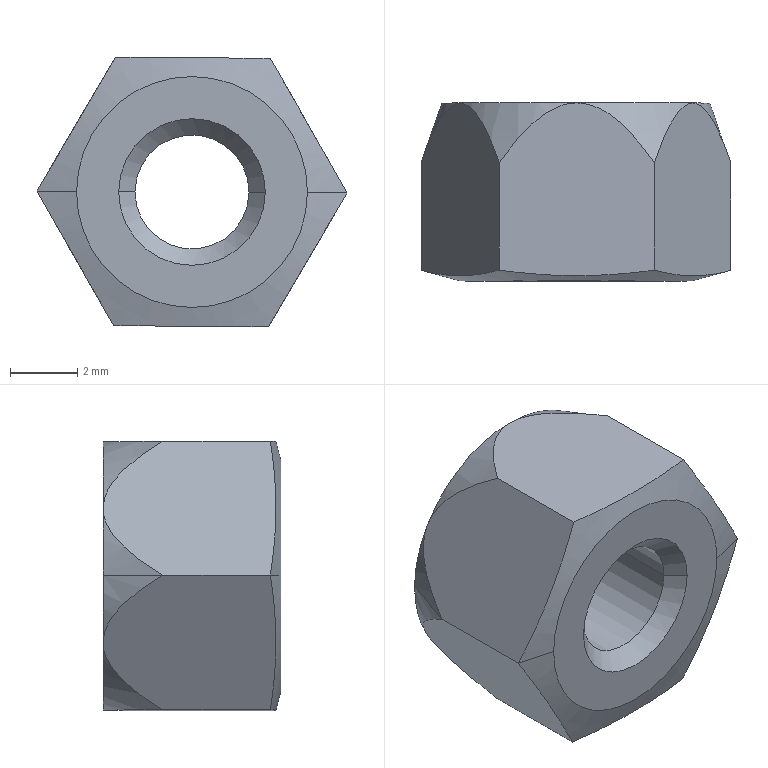Component | SolidWorks | prevailing torque all-metal 1 gb-4 | 1 solid | 21 faces | box 9.24 x 5.3 x 8.03 mm | volume 239 mm3 | cone 11 | plane 8 | cylinder 2 | commonest cylinder face diameters 3.4 x2
STEP:
#1=COLOUR_RGB('',0.7922,0.8196,0.9333);
#2=FILL_AREA_STYLE_COLOUR('',#1);
#3=FILL_AREA_STYLE('',(#2));
#4=SURFACE_STYLE_FILL_AREA(#3);
#5=SURFACE_SIDE_STYLE('',(#4));
#6=SURFACE_STYLE_USAGE(.BOTH.,#5);
#7=PRESENTATION_STYLE_ASSIGNMENT((#6));
#8=CARTESIAN_POINT('',(0.2638,-0.3076,1.348));
#9=VERTEX_POINT('',#8);
#10=CARTESIAN_POINT('',(0.1299,-0.3076,1.349));
#11=VERTEX_POINT('',#10);
#12=CARTESIAN_POINT('',(0.1969,-0.3076,1.348));
#13=DIRECTION('',(0.,-1.,0.));
#14=DIRECTION('',(-1.,0.,0.006451));
#15=AXIS2_PLACEMENT_3D('',#12,#13,#14);
#16=CIRCLE('',#15,0.06693);
#17=EDGE_CURVE('',#9,#11,#16,.T.);
#18=ORIENTED_EDGE('',*,*,#17,.F.);
#19=CARTESIAN_POINT('',(0.2829,-0.3268,1.348));
#20=VERTEX_POINT('',#19);
#21=CARTESIAN_POINT('',(0.2829,-0.3268,1.348));
#22=DIRECTION('',(0.7071,-0.7071,-0.004562));
#23=VECTOR('',#22,39.37);
#24=LINE('',#21,#23);
#25=EDGE_CURVE('',#9,#20,#24,.T.);
#26=ORIENTED_EDGE('',*,*,#25,.T.);
#27=CARTESIAN_POINT('',(0.1108,-0.3268,1.349));
#28=VERTEX_POINT('',#27);
#29=CARTESIAN_POINT('',(0.1969,-0.3268,1.348));
#30=DIRECTION('',(0.,1.,0.));
#31=DIRECTION('',(-1.,0.,0.006451));
#32=AXIS2_PLACEMENT_3D('',#29,#30,#31);
#33=CIRCLE('',#32,0.08605);
#34=EDGE_CURVE('',#28,#20,#33,.T.);
#35=ORIENTED_EDGE('',*,*,#34,.F.);
#36=CARTESIAN_POINT('',(0.1108,-0.3268,1.349));
#37=DIRECTION('',(-0.7071,-0.7071,0.004562));
#38=VECTOR('',#37,39.37);
#39=LINE('',#36,#38);
#40=EDGE_CURVE('',#11,#28,#39,.T.);
#41=ORIENTED_EDGE('',*,*,#40,.F.);
#42=EDGE_LOOP('',(#18,#26,#35,#41));
#43=FACE_OUTER_BOUND('',#42,.T.);
#44=CARTESIAN_POINT('',(0.1969,-0.3268,1.348));
#45=DIRECTION('',(0.,-1.,0.));
#46=DIRECTION('',(-1.,0.,0.006451));
#47=AXIS2_PLACEMENT_3D('',#44,#45,#46);
#48=CONICAL_SURFACE('',#47,0.08605,0.7854);
#49=ADVANCED_FACE('',(#43),#48,.F.);
#50=ORIENTED_EDGE('',*,*,#17,.T.);
#51=CARTESIAN_POINT('',(0.1299,-0.1181,1.349));
#52=VERTEX_POINT('',#51);
#53=CARTESIAN_POINT('',(0.1299,-0.3268,1.349));
#54=DIRECTION('',(0.,1.,0.));
#55=VECTOR('',#54,39.37);
#56=LINE('',#53,#55);
#57=EDGE_CURVE('',#11,#52,#56,.T.);
#58=ORIENTED_EDGE('',*,*,#57,.T.);
#59=CARTESIAN_POINT('',(0.2638,-0.1181,1.348));
#60=VERTEX_POINT('',#59);
#61=CARTESIAN_POINT('',(0.1969,-0.1181,1.348));
#62=DIRECTION('',(0.,1.,0.));
#63=DIRECTION('',(1.,0.,-0.006451));
#64=AXIS2_PLACEMENT_3D('',#61,#62,#63);
#65=CIRCLE('',#64,0.06693);
#66=EDGE_CURVE('',#52,#60,#65,.T.);
#67=ORIENTED_EDGE('',*,*,#66,.T.);
#68=CARTESIAN_POINT('',(0.2638,-0.3268,1.348));
#69=DIRECTION('',(0.,1.,0.));
#70=VECTOR('',#69,39.37);
#71=LINE('',#68,#70);
#72=EDGE_CURVE('',#9,#60,#71,.T.);
#73=ORIENTED_EDGE('',*,*,#72,.F.);
#74=EDGE_LOOP('',(#50,#58,#67,#73));
#75=FACE_OUTER_BOUND('',#74,.T.);
#76=CARTESIAN_POINT('',(0.1969,-0.3268,1.348));
#77=DIRECTION('',(0.,1.,0.));
#78=DIRECTION('',(1.,0.,-0.006451));
#79=AXIS2_PLACEMENT_3D('',#76,#77,#78);
#80=CYLINDRICAL_SURFACE('',#79,0.06693);
#81=ADVANCED_FACE('',(#75),#80,.F.);
#82=CARTESIAN_POINT('',(0.03937,-0.1181,1.349));
#83=VERTEX_POINT('',#82);
#84=CARTESIAN_POINT('',(0.06098,-0.1181,1.428));
#85=VERTEX_POINT('',#84);
#86=CARTESIAN_POINT('',(0.1969,-0.1181,1.348));
#87=DIRECTION('',(0.,1.,0.));
#88=DIRECTION('',(-1.,0.,0.006451));
#89=AXIS2_PLACEMENT_3D('',#86,#87,#88);
#90=CIRCLE('',#89,0.1575);
#91=EDGE_CURVE('',#83,#85,#90,.T.);
#92=ORIENTED_EDGE('',*,*,#91,.F.);
#93=CARTESIAN_POINT('',(0.01501,-0.1882,1.35));
#94=VERTEX_POINT('',#93);
#95=CARTESIAN_POINT('',(0.03937,-0.1181,1.349));
#96=DIRECTION('',(-0.3284,-0.9446,0.002118));
#97=VECTOR('',#96,39.37);
#98=LINE('',#95,#97);
#99=EDGE_CURVE('',#83,#94,#98,.T.);
#100=ORIENTED_EDGE('',*,*,#99,.T.);
#101=CARTESIAN_POINT('',(0.01501,-0.1882,1.35));
#102=CARTESIAN_POINT('',(0.01787,-0.18,1.354));
#103=CARTESIAN_POINT('',(0.02086,-0.1721,1.36));
#104=CARTESIAN_POINT('',(0.0272,-0.1569,1.37));
#105=CARTESIAN_POINT('',(0.03056,-0.1496,1.376));
#106=CARTESIAN_POINT('',(0.03795,-0.1363,1.389));
#107=CARTESIAN_POINT('',(0.042,-0.1301,1.396));
#108=CARTESIAN_POINT('',(0.05094,-0.121,1.411));
#109=CARTESIAN_POINT('',(0.05593,-0.1181,1.419));
#110=CARTESIAN_POINT('',(0.06098,-0.1181,1.428));
#111=B_SPLINE_CURVE_WITH_KNOTS('',3,(#101,#102,#103,#104,#105,#106,#107,#108,#109,#110),.UNSPECIFIED.,.F.,.F.,(4,2,2,2,4),(0.00000024,0.000751,0.001502,0.002252,0.003003),.UNSPECIFIED.);
#112=EDGE_CURVE('',#94,#85,#111,.T.);
#113=ORIENTED_EDGE('',*,*,#112,.T.);
#114=EDGE_LOOP('',(#92,#100,#113));
#115=FACE_OUTER_BOUND('',#114,.T.);
#116=CARTESIAN_POINT('',(0.1969,-0.1181,1.348));
#117=DIRECTION('',(0.,-1.,-0.));
#118=DIRECTION('',(-1.,-0.,0.006451));
#119=AXIS2_PLACEMENT_3D('',#116,#117,#118);
#120=CONICAL_SURFACE('',#119,0.1575,0.3346);
#121=ADVANCED_FACE('',(#115),#120,.T.);
#122=CARTESIAN_POINT('',(0.06142,-0.3268,1.349));
#123=VERTEX_POINT('',#122);
#124=CARTESIAN_POINT('',(0.3323,-0.3268,1.348));
#125=VERTEX_POINT('',#124);
#126=CARTESIAN_POINT('',(0.1969,-0.3268,1.348));
#127=DIRECTION('',(0.,-1.,-0.));
#128=DIRECTION('',(-1.,0.,0.006451));
#129=AXIS2_PLACEMENT_3D('',#126,#127,#128);
#130=CIRCLE('',#129,0.1354);
#131=EDGE_CURVE('',#123,#125,#130,.T.);
#132=ORIENTED_EDGE('',*,*,#131,.F.);
#133=CARTESIAN_POINT('',(0.01501,-0.3143,1.35));
#134=VERTEX_POINT('',#133);
#135=CARTESIAN_POINT('',(0.01501,-0.3143,1.35));
#136=DIRECTION('',(-0.9659,0.2588,0.006231));
#137=VECTOR('',#136,39.37);
#138=LINE('',#135,#137);
#139=EDGE_CURVE('',#123,#134,#138,.T.);
#140=ORIENTED_EDGE('',*,*,#139,.T.);
#141=CARTESIAN_POINT('',(0.1049,-0.3143,1.192));
#142=VERTEX_POINT('',#141);
#143=CARTESIAN_POINT('',(0.01501,-0.3143,1.35));
#144=CARTESIAN_POINT('',(0.03,-0.3184,1.323));
#145=CARTESIAN_POINT('',(0.05996,-0.3233,1.271));
#146=CARTESIAN_POINT('',(0.08993,-0.3184,1.218));
#147=CARTESIAN_POINT('',(0.1049,-0.3143,1.192));
#148=B_SPLINE_CURVE_WITH_KNOTS('',3,(#143,#144,#145,#146,#147),.UNSPECIFIED.,.F.,.F.,(4,1,4),(0.00000023,0.00231,0.004619),.UNSPECIFIED.);
#149=EDGE_CURVE('',#134,#142,#148,.T.);
#150=ORIENTED_EDGE('',*,*,#149,.T.);
#151=CARTESIAN_POINT('',(0.2868,-0.3143,1.19));
#152=VERTEX_POINT('',#151);
#153=CARTESIAN_POINT('',(0.1049,-0.3143,1.192));
#154=CARTESIAN_POINT('',(0.12,-0.3164,1.191));
#155=CARTESIAN_POINT('',(0.1353,-0.318,1.191));
#156=CARTESIAN_POINT('',(0.1657,-0.3203,1.191));
#157=CARTESIAN_POINT('',(0.1808,-0.3209,1.191));
#158=CARTESIAN_POINT('',(0.2263,-0.3209,1.191));
#159=CARTESIAN_POINT('',(0.2566,-0.3184,1.191));
#160=CARTESIAN_POINT('',(0.2868,-0.3143,1.19));
#161=B_SPLINE_CURVE_WITH_KNOTS('',3,(#153,#154,#155,#156,#157,#158,#159,#160),.UNSPECIFIED.,.F.,.F.,(4,2,2,4),(0.003852,0.005015,0.006177,0.008501),.UNSPECIFIED.);
#162=EDGE_CURVE('',#142,#152,#161,.T.);
#163=ORIENTED_EDGE('',*,*,#162,.T.);
#164=CARTESIAN_POINT('',(0.3787,-0.3143,1.347));
#165=VERTEX_POINT('',#164);
#166=CARTESIAN_POINT('',(0.2868,-0.3143,1.19));
#167=CARTESIAN_POINT('',(0.3021,-0.3184,1.217));
#168=CARTESIAN_POINT('',(0.3327,-0.3233,1.269));
#169=CARTESIAN_POINT('',(0.3634,-0.3184,1.321));
#170=CARTESIAN_POINT('',(0.3787,-0.3143,1.347));
#171=B_SPLINE_CURVE_WITH_KNOTS('',3,(#166,#167,#168,#169,#170),.UNSPECIFIED.,.F.,.F.,(4,1,4),(0.00000023,0.00231,0.004619),.UNSPECIFIED.);
#172=EDGE_CURVE('',#152,#165,#171,.T.);
#173=ORIENTED_EDGE('',*,*,#172,.T.);
#174=CARTESIAN_POINT('',(0.3787,-0.3143,1.347));
#175=DIRECTION('',(0.9659,0.2588,-0.006231));
#176=VECTOR('',#175,39.37);
#177=LINE('',#174,#176);
#178=EDGE_CURVE('',#125,#165,#177,.T.);
#179=ORIENTED_EDGE('',*,*,#178,.F.);
#180=EDGE_LOOP('',(#132,#140,#150,#163,#173,#179));
#181=FACE_OUTER_BOUND('',#180,.T.);
#182=CARTESIAN_POINT('',(0.1969,-0.3143,1.348));
#183=DIRECTION('',(-0.,1.,0.));
#184=DIRECTION('',(1.,0.,-0.006451));
#185=AXIS2_PLACEMENT_3D('',#182,#183,#184);
#186=CONICAL_SURFACE('',#185,0.1818,1.309);
#187=ADVANCED_FACE('',(#181),#186,.T.);
#188=CARTESIAN_POINT('',(0.1069,-0.1882,1.506));
#189=VERTEX_POINT('',#188);
#190=CARTESIAN_POINT('',(0.1979,-0.1181,1.506));
#191=VERTEX_POINT('',#190);
#192=CARTESIAN_POINT('',(0.1069,-0.1882,1.506));
#193=CARTESIAN_POINT('',(0.1126,-0.1801,1.506));
#194=CARTESIAN_POINT('',(0.1184,-0.1722,1.506));
#195=CARTESIAN_POINT('',(0.131,-0.157,1.506));
#196=CARTESIAN_POINT('',(0.1378,-0.1496,1.506));
#197=CARTESIAN_POINT('',(0.1524,-0.1362,1.506));
#198=CARTESIAN_POINT('',(0.1604,-0.1301,1.506));
#199=CARTESIAN_POINT('',(0.1737,-0.1233,1.506));
#200=CARTESIAN_POINT('',(0.1783,-0.1214,1.506));
#201=CARTESIAN_POINT('',(0.188,-0.1188,1.506));
#202=CARTESIAN_POINT('',(0.1929,-0.1181,1.506));
#203=CARTESIAN_POINT('',(0.1979,-0.1181,1.506));
#204=B_SPLINE_CURVE_WITH_KNOTS('',3,(#192,#193,#194,#195,#196,#197,#198,#199,#200,#201,#202,#203),.UNSPECIFIED.,.F.,.F.,(4,2,2,2,2,4),(0.003325,0.004072,0.004819,0.005566,0.00594,0.006313),.UNSPECIFIED.);
#205=EDGE_CURVE('',#189,#191,#204,.T.);
#206=ORIENTED_EDGE('',*,*,#205,.F.);
#207=CARTESIAN_POINT('',(0.1069,-0.3143,1.506));
#208=VERTEX_POINT('',#207);
#209=CARTESIAN_POINT('',(0.1069,-0.3268,1.506));
#210=DIRECTION('',(0.,1.,0.));
#211=VECTOR('',#210,39.37);
#212=LINE('',#209,#211);
#213=EDGE_CURVE('',#208,#189,#212,.T.);
#214=ORIENTED_EDGE('',*,*,#213,.F.);
#215=CARTESIAN_POINT('',(0.2888,-0.3143,1.505));
#216=VERTEX_POINT('',#215);
#217=CARTESIAN_POINT('',(0.2888,-0.3143,1.505));
#218=CARTESIAN_POINT('',(0.2586,-0.3184,1.506));
#219=CARTESIAN_POINT('',(0.2283,-0.3209,1.506));
#220=CARTESIAN_POINT('',(0.1829,-0.3209,1.506));
#221=CARTESIAN_POINT('',(0.1677,-0.3203,1.506));
#222=CARTESIAN_POINT('',(0.1373,-0.318,1.506));
#223=CARTESIAN_POINT('',(0.1221,-0.3164,1.506));
#224=CARTESIAN_POINT('',(0.1069,-0.3143,1.506));
#225=B_SPLINE_CURVE_WITH_KNOTS('',3,(#217,#218,#219,#220,#221,#222,#223,#224),.UNSPECIFIED.,.F.,.F.,(4,2,2,4),(0.008829,0.01115,0.01231,0.01347),.UNSPECIFIED.);
#226=EDGE_CURVE('',#216,#208,#225,.T.);
#227=ORIENTED_EDGE('',*,*,#226,.F.);
#228=CARTESIAN_POINT('',(0.2888,-0.1882,1.505));
#229=VERTEX_POINT('',#228);
#230=CARTESIAN_POINT('',(0.2888,-0.3268,1.505));
#231=DIRECTION('',(0.,1.,0.));
#232=VECTOR('',#231,39.37);
#233=LINE('',#230,#232);
#234=EDGE_CURVE('',#216,#229,#233,.T.);
#235=ORIENTED_EDGE('',*,*,#234,.T.);
#236=CARTESIAN_POINT('',(0.1979,-0.1181,1.506));
#237=CARTESIAN_POINT('',(0.2079,-0.1181,1.506));
#238=CARTESIAN_POINT('',(0.2178,-0.121,1.506));
#239=CARTESIAN_POINT('',(0.2354,-0.1301,1.506));
#240=CARTESIAN_POINT('',(0.2434,-0.1363,1.506));
#241=CARTESIAN_POINT('',(0.258,-0.1497,1.506));
#242=CARTESIAN_POINT('',(0.2647,-0.1569,1.505));
#243=CARTESIAN_POINT('',(0.2772,-0.1721,1.505));
#244=CARTESIAN_POINT('',(0.2831,-0.18,1.505));
#245=CARTESIAN_POINT('',(0.2888,-0.1882,1.505));
#246=B_SPLINE_CURVE_WITH_KNOTS('',3,(#236,#237,#238,#239,#240,#241,#242,#243,#244,#245),.UNSPECIFIED.,.F.,.F.,(4,2,2,2,4),(0.006313,0.007062,0.007811,0.00856,0.009309),.UNSPECIFIED.);
#247=EDGE_CURVE('',#191,#229,#246,.T.);
#248=ORIENTED_EDGE('',*,*,#247,.F.);
#249=EDGE_LOOP('',(#206,#214,#227,#235,#248));
#250=FACE_OUTER_BOUND('',#249,.T.);
#251=CARTESIAN_POINT('',(0.1069,-0.3268,1.506));
#252=DIRECTION('',(0.006451,0.,1.));
#253=DIRECTION('',(0.,-1.,0.));
#254=AXIS2_PLACEMENT_3D('',#251,#252,#253);
#255=PLANE('',#254);
#256=ADVANCED_FACE('',(#250),#255,.T.);
#257=ORIENTED_EDGE('',*,*,#112,.F.);
#258=CARTESIAN_POINT('',(0.01501,-0.3268,1.35));
#259=DIRECTION('',(0.,1.,0.));
#260=VECTOR('',#259,39.37);
#261=LINE('',#258,#260);
#262=EDGE_CURVE('',#134,#94,#261,.T.);
#263=ORIENTED_EDGE('',*,*,#262,.F.);
#264=CARTESIAN_POINT('',(0.1069,-0.3143,1.506));
#265=CARTESIAN_POINT('',(0.09162,-0.3184,1.48));
#266=CARTESIAN_POINT('',(0.06098,-0.3233,1.428));
#267=CARTESIAN_POINT('',(0.03033,-0.3184,1.376));
#268=CARTESIAN_POINT('',(0.01501,-0.3143,1.35));
#269=B_SPLINE_CURVE_WITH_KNOTS('',3,(#264,#265,#266,#267,#268),.UNSPECIFIED.,.F.,.F.,(4,1,4),(0.00000023,0.00231,0.004619),.UNSPECIFIED.);
#270=EDGE_CURVE('',#208,#134,#269,.T.);
#271=ORIENTED_EDGE('',*,*,#270,.F.);
#272=ORIENTED_EDGE('',*,*,#213,.T.);
#273=CARTESIAN_POINT('',(0.06098,-0.1181,1.428));
#274=CARTESIAN_POINT('',(0.06602,-0.1181,1.437));
#275=CARTESIAN_POINT('',(0.07098,-0.121,1.445));
#276=CARTESIAN_POINT('',(0.07988,-0.13,1.46));
#277=CARTESIAN_POINT('',(0.08394,-0.1362,1.467));
#278=CARTESIAN_POINT('',(0.09131,-0.1495,1.48));
#279=CARTESIAN_POINT('',(0.09469,-0.1568,1.486));
#280=CARTESIAN_POINT('',(0.1011,-0.1721,1.496));
#281=CARTESIAN_POINT('',(0.1041,-0.18,1.502));
#282=CARTESIAN_POINT('',(0.1069,-0.1882,1.506));
#283=B_SPLINE_CURVE_WITH_KNOTS('',3,(#273,#274,#275,#276,#277,#278,#279,#280,#281,#282),.UNSPECIFIED.,.F.,.F.,(4,2,2,2,4),(0.003003,0.003753,0.004503,0.005252,0.006002),.UNSPECIFIED.);
#284=EDGE_CURVE('',#85,#189,#283,.T.);
#285=ORIENTED_EDGE('',*,*,#284,.F.);
#286=EDGE_LOOP('',(#257,#263,#271,#272,#285));
#287=FACE_OUTER_BOUND('',#286,.T.);
#288=CARTESIAN_POINT('',(0.01501,-0.3268,1.35));
#289=DIRECTION('',(-0.8628,0.,0.5056));
#290=DIRECTION('',(0.5056,0.,0.8628));
#291=AXIS2_PLACEMENT_3D('',#288,#289,#290);
#292=PLANE('',#291);
#293=ADVANCED_FACE('',(#287),#292,.T.);
#294=CARTESIAN_POINT('',(0.1049,-0.1882,1.192));
#295=VERTEX_POINT('',#294);
#296=CARTESIAN_POINT('',(0.05996,-0.1181,1.271));
#297=VERTEX_POINT('',#296);
#298=CARTESIAN_POINT('',(0.1049,-0.1882,1.192));
#299=CARTESIAN_POINT('',(0.1021,-0.18,1.196));
#300=CARTESIAN_POINT('',(0.0992,-0.1721,1.202));
#301=CARTESIAN_POINT('',(0.09299,-0.1569,1.212));
#302=CARTESIAN_POINT('',(0.08971,-0.1496,1.218));
#303=CARTESIAN_POINT('',(0.08248,-0.1363,1.231));
#304=CARTESIAN_POINT('',(0.07852,-0.1301,1.238));
#305=CARTESIAN_POINT('',(0.06978,-0.121,1.253));
#306=CARTESIAN_POINT('',(0.0649,-0.1181,1.262));
#307=CARTESIAN_POINT('',(0.05996,-0.1181,1.271));
#308=B_SPLINE_CURVE_WITH_KNOTS('',3,(#298,#299,#300,#301,#302,#303,#304,#305,#306,#307),.UNSPECIFIED.,.F.,.F.,(4,2,2,2,4),(0.00000024,0.000751,0.001502,0.002252,0.003003),.UNSPECIFIED.);
#309=EDGE_CURVE('',#295,#297,#308,.T.);
#310=ORIENTED_EDGE('',*,*,#309,.F.);
#311=CARTESIAN_POINT('',(0.1049,-0.3268,1.192));
#312=DIRECTION('',(0.,1.,0.));
#313=VECTOR('',#312,39.37);
#314=LINE('',#311,#313);
#315=EDGE_CURVE('',#142,#295,#314,.T.);
#316=ORIENTED_EDGE('',*,*,#315,.F.);
#317=ORIENTED_EDGE('',*,*,#149,.F.);
#318=ORIENTED_EDGE('',*,*,#262,.T.);
#319=CARTESIAN_POINT('',(0.05996,-0.1181,1.271));
#320=CARTESIAN_POINT('',(0.05503,-0.1181,1.279));
#321=CARTESIAN_POINT('',(0.05018,-0.121,1.288));
#322=CARTESIAN_POINT('',(0.04148,-0.13,1.303));
#323=CARTESIAN_POINT('',(0.03751,-0.1362,1.31));
#324=CARTESIAN_POINT('',(0.0303,-0.1495,1.323));
#325=CARTESIAN_POINT('',(0.027,-0.1568,1.329));
#326=CARTESIAN_POINT('',(0.02075,-0.1721,1.34));
#327=CARTESIAN_POINT('',(0.01781,-0.18,1.345));
#328=CARTESIAN_POINT('',(0.01501,-0.1882,1.35));
#329=B_SPLINE_CURVE_WITH_KNOTS('',3,(#319,#320,#321,#322,#323,#324,#325,#326,#327,#328),.UNSPECIFIED.,.F.,.F.,(4,2,2,2,4),(0.003003,0.003753,0.004503,0.005252,0.006002),.UNSPECIFIED.);
#330=EDGE_CURVE('',#297,#94,#329,.T.);
#331=ORIENTED_EDGE('',*,*,#330,.F.);
#332=EDGE_LOOP('',(#310,#316,#317,#318,#331));
#333=FACE_OUTER_BOUND('',#332,.T.);
#334=CARTESIAN_POINT('',(0.1049,-0.3268,1.192));
#335=DIRECTION('',(-0.8692,0.,-0.4944));
#336=DIRECTION('',(-0.4944,0.,0.8692));
#337=AXIS2_PLACEMENT_3D('',#334,#335,#336);
#338=PLANE('',#337);
#339=ADVANCED_FACE('',(#333),#338,.T.);
#340=CARTESIAN_POINT('',(0.2868,-0.1882,1.19));
#341=VERTEX_POINT('',#340);
#342=CARTESIAN_POINT('',(0.1958,-0.1181,1.191));
#343=VERTEX_POINT('',#342);
#344=CARTESIAN_POINT('',(0.2868,-0.1882,1.19));
#345=CARTESIAN_POINT('',(0.2811,-0.18,1.19));
#346=CARTESIAN_POINT('',(0.2752,-0.1721,1.19));
#347=CARTESIAN_POINT('',(0.2627,-0.1569,1.191));
#348=CARTESIAN_POINT('',(0.256,-0.1497,1.191));
#349=CARTESIAN_POINT('',(0.2414,-0.1363,1.191));
#350=CARTESIAN_POINT('',(0.2334,-0.1301,1.191));
#351=CARTESIAN_POINT('',(0.2157,-0.121,1.191));
#352=CARTESIAN_POINT('',(0.2059,-0.1181,1.191));
#353=CARTESIAN_POINT('',(0.1958,-0.1181,1.191));
#354=B_SPLINE_CURVE_WITH_KNOTS('',3,(#344,#345,#346,#347,#348,#349,#350,#351,#352,#353),.UNSPECIFIED.,.F.,.F.,(4,2,2,2,4),(0.008014,0.008762,0.00951,0.01026,0.01101),.UNSPECIFIED.);
#355=EDGE_CURVE('',#341,#343,#354,.T.);
#356=ORIENTED_EDGE('',*,*,#355,.F.);
#357=CARTESIAN_POINT('',(0.2868,-0.3268,1.19));
#358=DIRECTION('',(0.,1.,0.));
#359=VECTOR('',#358,39.37);
#360=LINE('',#357,#359);
#361=EDGE_CURVE('',#152,#341,#360,.T.);
#362=ORIENTED_EDGE('',*,*,#361,.F.);
#363=ORIENTED_EDGE('',*,*,#162,.F.);
#364=ORIENTED_EDGE('',*,*,#315,.T.);
#365=CARTESIAN_POINT('',(0.1958,-0.1181,1.191));
#366=CARTESIAN_POINT('',(0.1908,-0.1181,1.191));
#367=CARTESIAN_POINT('',(0.1859,-0.1188,1.191));
#368=CARTESIAN_POINT('',(0.1763,-0.1214,1.191));
#369=CARTESIAN_POINT('',(0.1716,-0.1233,1.191));
#370=CARTESIAN_POINT('',(0.1584,-0.1301,1.191));
#371=CARTESIAN_POINT('',(0.1504,-0.1362,1.191));
#372=CARTESIAN_POINT('',(0.1357,-0.1496,1.191));
#373=CARTESIAN_POINT('',(0.129,-0.157,1.191));
#374=CARTESIAN_POINT('',(0.1164,-0.1722,1.191));
#375=CARTESIAN_POINT('',(0.1105,-0.1801,1.191));
#376=CARTESIAN_POINT('',(0.1049,-0.1882,1.192));
#377=B_SPLINE_CURVE_WITH_KNOTS('',3,(#365,#366,#367,#368,#369,#370,#371,#372,#373,#374,#375,#376),.UNSPECIFIED.,.F.,.F.,(4,2,2,2,2,4),(0.01101,0.01138,0.01175,0.0125,0.01324,0.01399),.UNSPECIFIED.);
#378=EDGE_CURVE('',#343,#295,#377,.T.);
#379=ORIENTED_EDGE('',*,*,#378,.F.);
#380=EDGE_LOOP('',(#356,#362,#363,#364,#379));
#381=FACE_OUTER_BOUND('',#380,.T.);
#382=CARTESIAN_POINT('',(0.2868,-0.3268,1.19));
#383=DIRECTION('',(-0.006451,0.,-1.));
#384=DIRECTION('',(0.,1.,0.));
#385=AXIS2_PLACEMENT_3D('',#382,#383,#384);
#386=PLANE('',#385);
#387=ADVANCED_FACE('',(#381),#386,.T.);
#388=CARTESIAN_POINT('',(0.3787,-0.1882,1.347));
#389=VERTEX_POINT('',#388);
#390=CARTESIAN_POINT('',(0.3327,-0.1181,1.269));
#391=VERTEX_POINT('',#390);
#392=CARTESIAN_POINT('',(0.3787,-0.1882,1.347));
#393=CARTESIAN_POINT('',(0.3758,-0.18,1.342));
#394=CARTESIAN_POINT('',(0.3728,-0.1721,1.337));
#395=CARTESIAN_POINT('',(0.3665,-0.1569,1.326));
#396=CARTESIAN_POINT('',(0.3631,-0.1496,1.321));
#397=CARTESIAN_POINT('',(0.3557,-0.1363,1.308));
#398=CARTESIAN_POINT('',(0.3517,-0.1301,1.301));
#399=CARTESIAN_POINT('',(0.3428,-0.121,1.286));
#400=CARTESIAN_POINT('',(0.3378,-0.1181,1.277));
#401=CARTESIAN_POINT('',(0.3327,-0.1181,1.269));
#402=B_SPLINE_CURVE_WITH_KNOTS('',3,(#392,#393,#394,#395,#396,#397,#398,#399,#400,#401),.UNSPECIFIED.,.F.,.F.,(4,2,2,2,4),(0.00000024,0.000751,0.001502,0.002252,0.003003),.UNSPECIFIED.);
#403=EDGE_CURVE('',#389,#391,#402,.T.);
#404=ORIENTED_EDGE('',*,*,#403,.F.);
#405=CARTESIAN_POINT('',(0.3787,-0.3268,1.347));
#406=DIRECTION('',(0.,1.,0.));
#407=VECTOR('',#406,39.37);
#408=LINE('',#405,#407);
#409=EDGE_CURVE('',#165,#389,#408,.T.);
#410=ORIENTED_EDGE('',*,*,#409,.F.);
#411=ORIENTED_EDGE('',*,*,#172,.F.);
#412=ORIENTED_EDGE('',*,*,#361,.T.);
#413=CARTESIAN_POINT('',(0.3327,-0.1181,1.269));
#414=CARTESIAN_POINT('',(0.3277,-0.1181,1.26));
#415=CARTESIAN_POINT('',(0.3227,-0.121,1.252));
#416=CARTESIAN_POINT('',(0.3138,-0.13,1.237));
#417=CARTESIAN_POINT('',(0.3098,-0.1362,1.23));
#418=CARTESIAN_POINT('',(0.3024,-0.1495,1.217));
#419=CARTESIAN_POINT('',(0.299,-0.1568,1.211));
#420=CARTESIAN_POINT('',(0.2926,-0.1721,1.2));
#421=CARTESIAN_POINT('',(0.2896,-0.18,1.195));
#422=CARTESIAN_POINT('',(0.2868,-0.1882,1.19));
#423=B_SPLINE_CURVE_WITH_KNOTS('',3,(#413,#414,#415,#416,#417,#418,#419,#420,#421,#422),.UNSPECIFIED.,.F.,.F.,(4,2,2,2,4),(0.003003,0.003753,0.004503,0.005252,0.006002),.UNSPECIFIED.);
#424=EDGE_CURVE('',#391,#341,#423,.T.);
#425=ORIENTED_EDGE('',*,*,#424,.F.);
#426=EDGE_LOOP('',(#404,#410,#411,#412,#425));
#427=FACE_OUTER_BOUND('',#426,.T.);
#428=CARTESIAN_POINT('',(0.3787,-0.3268,1.347));
#429=DIRECTION('',(0.8628,0.,-0.5056));
#430=DIRECTION('',(-0.5056,0.,-0.8628));
#431=AXIS2_PLACEMENT_3D('',#428,#429,#430);
#432=PLANE('',#431);
#433=ADVANCED_FACE('',(#427),#432,.T.);
#434=CARTESIAN_POINT('',(0.3337,-0.1181,1.426));
#435=VERTEX_POINT('',#434);
#436=CARTESIAN_POINT('',(0.2888,-0.1882,1.505));
#437=CARTESIAN_POINT('',(0.2916,-0.18,1.5));
#438=CARTESIAN_POINT('',(0.2945,-0.1721,1.495));
#439=CARTESIAN_POINT('',(0.3007,-0.1569,1.484));
#440=CARTESIAN_POINT('',(0.304,-0.1496,1.479));
#441=CARTESIAN_POINT('',(0.3112,-0.1363,1.466));
#442=CARTESIAN_POINT('',(0.3152,-0.1301,1.459));
#443=CARTESIAN_POINT('',(0.3239,-0.121,1.444));
#444=CARTESIAN_POINT('',(0.3288,-0.1181,1.435));
#445=CARTESIAN_POINT('',(0.3337,-0.1181,1.426));
#446=B_SPLINE_CURVE_WITH_KNOTS('',3,(#436,#437,#438,#439,#440,#441,#442,#443,#444,#445),.UNSPECIFIED.,.F.,.F.,(4,2,2,2,4),(0.00000024,0.000751,0.001502,0.002252,0.003003),.UNSPECIFIED.);
#447=EDGE_CURVE('',#229,#435,#446,.T.);
#448=ORIENTED_EDGE('',*,*,#447,.F.);
#449=ORIENTED_EDGE('',*,*,#234,.F.);
#450=CARTESIAN_POINT('',(0.3787,-0.3143,1.347));
#451=CARTESIAN_POINT('',(0.3637,-0.3184,1.374));
#452=CARTESIAN_POINT('',(0.3337,-0.3233,1.426));
#453=CARTESIAN_POINT('',(0.3038,-0.3184,1.479));
#454=CARTESIAN_POINT('',(0.2888,-0.3143,1.505));
#455=B_SPLINE_CURVE_WITH_KNOTS('',3,(#450,#451,#452,#453,#454),.UNSPECIFIED.,.F.,.F.,(4,1,4),(0.00000023,0.00231,0.004619),.UNSPECIFIED.);
#456=EDGE_CURVE('',#165,#216,#455,.T.);
#457=ORIENTED_EDGE('',*,*,#456,.F.);
#458=ORIENTED_EDGE('',*,*,#409,.T.);
#459=CARTESIAN_POINT('',(0.3337,-0.1181,1.426));
#460=CARTESIAN_POINT('',(0.3387,-0.1181,1.418));
#461=CARTESIAN_POINT('',(0.3435,-0.121,1.409));
#462=CARTESIAN_POINT('',(0.3522,-0.13,1.394));
#463=CARTESIAN_POINT('',(0.3562,-0.1362,1.387));
#464=CARTESIAN_POINT('',(0.3634,-0.1495,1.374));
#465=CARTESIAN_POINT('',(0.3667,-0.1568,1.368));
#466=CARTESIAN_POINT('',(0.373,-0.1721,1.357));
#467=CARTESIAN_POINT('',(0.3759,-0.18,1.352));
#468=CARTESIAN_POINT('',(0.3787,-0.1882,1.347));
#469=B_SPLINE_CURVE_WITH_KNOTS('',3,(#459,#460,#461,#462,#463,#464,#465,#466,#467,#468),.UNSPECIFIED.,.F.,.F.,(4,2,2,2,4),(0.003003,0.003753,0.004503,0.005252,0.006002),.UNSPECIFIED.);
#470=EDGE_CURVE('',#435,#389,#469,.T.);
#471=ORIENTED_EDGE('',*,*,#470,.F.);
#472=EDGE_LOOP('',(#448,#449,#457,#458,#471));
#473=FACE_OUTER_BOUND('',#472,.T.);
#474=CARTESIAN_POINT('',(0.2888,-0.3268,1.505));
#475=DIRECTION('',(0.8692,0.,0.4944));
#476=DIRECTION('',(0.4944,0.,-0.8692));
#477=AXIS2_PLACEMENT_3D('',#474,#475,#476);
#478=PLANE('',#477);
#479=ADVANCED_FACE('',(#473),#478,.T.);
#480=ORIENTED_EDGE('',*,*,#139,.F.);
#481=CARTESIAN_POINT('',(0.1969,-0.3268,1.348));
#482=DIRECTION('',(0.,-1.,-0.));
#483=DIRECTION('',(-1.,0.,0.006451));
#484=AXIS2_PLACEMENT_3D('',#481,#482,#483);
#485=CIRCLE('',#484,0.1354);
#486=EDGE_CURVE('',#125,#123,#485,.T.);
#487=ORIENTED_EDGE('',*,*,#486,.F.);
#488=ORIENTED_EDGE('',*,*,#178,.T.);
#489=ORIENTED_EDGE('',*,*,#456,.T.);
#490=ORIENTED_EDGE('',*,*,#226,.T.);
#491=ORIENTED_EDGE('',*,*,#270,.T.);
#492=EDGE_LOOP('',(#480,#487,#488,#489,#490,#491));
#493=FACE_OUTER_BOUND('',#492,.T.);
#494=CARTESIAN_POINT('',(0.1969,-0.3143,1.348));
#495=DIRECTION('',(-0.,1.,0.));
#496=DIRECTION('',(1.,0.,-0.006451));
#497=AXIS2_PLACEMENT_3D('',#494,#495,#496);
#498=CONICAL_SURFACE('',#497,0.1818,1.309);
#499=ADVANCED_FACE('',(#493),#498,.T.);
#500=ORIENTED_EDGE('',*,*,#34,.T.);
#501=CARTESIAN_POINT('',(0.1969,-0.3268,1.348));
#502=DIRECTION('',(0.,1.,0.));
#503=DIRECTION('',(-1.,0.,0.006451));
#504=AXIS2_PLACEMENT_3D('',#501,#502,#503);
#505=CIRCLE('',#504,0.08605);
#506=EDGE_CURVE('',#20,#28,#505,.T.);
#507=ORIENTED_EDGE('',*,*,#506,.T.);
#508=EDGE_LOOP('',(#500,#507));
#509=FACE_BOUND('',#508,.T.);
#510=ORIENTED_EDGE('',*,*,#486,.T.);
#511=ORIENTED_EDGE('',*,*,#131,.T.);
#512=EDGE_LOOP('',(#510,#511));
#513=FACE_OUTER_BOUND('',#512,.T.);
#514=CARTESIAN_POINT('',(0.1069,-0.3268,1.506));
#515=DIRECTION('',(0.,-1.,0.));
#516=DIRECTION('',(-1.,0.,0.006451));
#517=AXIS2_PLACEMENT_3D('',#514,#515,#516);
#518=PLANE('',#517);
#519=ADVANCED_FACE('',(#509,#513),#518,.T.);
#520=ORIENTED_EDGE('',*,*,#99,.F.);
#521=CARTESIAN_POINT('',(0.1969,-0.1181,1.348));
#522=DIRECTION('',(0.,1.,0.));
#523=DIRECTION('',(-1.,0.,0.006451));
#524=AXIS2_PLACEMENT_3D('',#521,#522,#523);
#525=CIRCLE('',#524,0.1575);
#526=EDGE_CURVE('',#297,#83,#525,.T.);
#527=ORIENTED_EDGE('',*,*,#526,.F.);
#528=ORIENTED_EDGE('',*,*,#330,.T.);
#529=EDGE_LOOP('',(#520,#527,#528));
#530=FACE_OUTER_BOUND('',#529,.T.);
#531=CARTESIAN_POINT('',(0.1969,-0.1181,1.348));
#532=DIRECTION('',(0.,-1.,-0.));
#533=DIRECTION('',(-1.,-0.,0.006451));
#534=AXIS2_PLACEMENT_3D('',#531,#532,#533);
#535=CONICAL_SURFACE('',#534,0.1575,0.3346);
#536=ADVANCED_FACE('',(#530),#535,.T.);
#537=ORIENTED_EDGE('',*,*,#309,.T.);
#538=CARTESIAN_POINT('',(0.1969,-0.1181,1.348));
#539=DIRECTION('',(0.,-1.,-0.));
#540=DIRECTION('',(-1.,-0.,0.006451));
#541=AXIS2_PLACEMENT_3D('',#538,#539,#540);
#542=CIRCLE('',#541,0.1575);
#543=EDGE_CURVE('',#297,#343,#542,.T.);
#544=ORIENTED_EDGE('',*,*,#543,.T.);
#545=ORIENTED_EDGE('',*,*,#378,.T.);
#546=EDGE_LOOP('',(#537,#544,#545));
#547=FACE_OUTER_BOUND('',#546,.T.);
#548=CARTESIAN_POINT('',(0.1969,-0.1181,1.348));
#549=DIRECTION('',(0.,-1.,-0.));
#550=DIRECTION('',(-1.,-0.,0.006451));
#551=AXIS2_PLACEMENT_3D('',#548,#549,#550);
#552=CONICAL_SURFACE('',#551,0.1575,0.3346);
#553=ADVANCED_FACE('',(#547),#552,.T.);
#554=ORIENTED_EDGE('',*,*,#355,.T.);
#555=CARTESIAN_POINT('',(0.1969,-0.1181,1.348));
#556=DIRECTION('',(0.,1.,0.));
#557=DIRECTION('',(-1.,0.,0.006451));
#558=AXIS2_PLACEMENT_3D('',#555,#556,#557);
#559=CIRCLE('',#558,0.1575);
#560=EDGE_CURVE('',#391,#343,#559,.T.);
#561=ORIENTED_EDGE('',*,*,#560,.F.);
#562=ORIENTED_EDGE('',*,*,#424,.T.);
#563=EDGE_LOOP('',(#554,#561,#562));
#564=FACE_OUTER_BOUND('',#563,.T.);
#565=CARTESIAN_POINT('',(0.1969,-0.1181,1.348));
#566=DIRECTION('',(0.,-1.,-0.));
#567=DIRECTION('',(-1.,-0.,0.006451));
#568=AXIS2_PLACEMENT_3D('',#565,#566,#567);
#569=CONICAL_SURFACE('',#568,0.1575,0.3346);
#570=ADVANCED_FACE('',(#564),#569,.T.);
#571=ORIENTED_EDGE('',*,*,#403,.T.);
#572=CARTESIAN_POINT('',(0.1969,-0.1181,1.348));
#573=DIRECTION('',(0.,1.,0.));
#574=DIRECTION('',(-1.,0.,0.006451));
#575=AXIS2_PLACEMENT_3D('',#572,#573,#574);
#576=CIRCLE('',#575,0.1575);
#577=EDGE_CURVE('',#435,#391,#576,.T.);
#578=ORIENTED_EDGE('',*,*,#577,.F.);
#579=ORIENTED_EDGE('',*,*,#470,.T.);
#580=EDGE_LOOP('',(#571,#578,#579));
#581=FACE_OUTER_BOUND('',#580,.T.);
#582=CARTESIAN_POINT('',(0.1969,-0.1181,1.348));
#583=DIRECTION('',(0.,-1.,-0.));
#584=DIRECTION('',(-1.,-0.,0.006451));
#585=AXIS2_PLACEMENT_3D('',#582,#583,#584);
#586=CONICAL_SURFACE('',#585,0.1575,0.3346);
#587=ADVANCED_FACE('',(#581),#586,.T.);
#588=ORIENTED_EDGE('',*,*,#247,.T.);
#589=ORIENTED_EDGE('',*,*,#447,.T.);
#590=CARTESIAN_POINT('',(0.1969,-0.1181,1.348));
#591=DIRECTION('',(0.,1.,0.));
#592=DIRECTION('',(-1.,0.,0.006451));
#593=AXIS2_PLACEMENT_3D('',#590,#591,#592);
#594=CIRCLE('',#593,0.1575);
#595=EDGE_CURVE('',#191,#435,#594,.T.);
#596=ORIENTED_EDGE('',*,*,#595,.F.);
#597=EDGE_LOOP('',(#588,#589,#596));
#598=FACE_OUTER_BOUND('',#597,.T.);
#599=CARTESIAN_POINT('',(0.1969,-0.1181,1.348));
#600=DIRECTION('',(0.,-1.,-0.));
#601=DIRECTION('',(-1.,-0.,0.006451));
#602=AXIS2_PLACEMENT_3D('',#599,#600,#601);
#603=CONICAL_SURFACE('',#602,0.1575,0.3346);
#604=ADVANCED_FACE('',(#598),#603,.T.);
#605=ORIENTED_EDGE('',*,*,#284,.T.);
#606=ORIENTED_EDGE('',*,*,#205,.T.);
#607=CARTESIAN_POINT('',(0.1969,-0.1181,1.348));
#608=DIRECTION('',(0.,1.,0.));
#609=DIRECTION('',(-1.,0.,0.006451));
#610=AXIS2_PLACEMENT_3D('',#607,#608,#609);
#611=CIRCLE('',#610,0.1575);
#612=EDGE_CURVE('',#85,#191,#611,.T.);
#613=ORIENTED_EDGE('',*,*,#612,.F.);
#614=EDGE_LOOP('',(#605,#606,#613));
#615=FACE_OUTER_BOUND('',#614,.T.);
#616=CARTESIAN_POINT('',(0.1969,-0.1181,1.348));
#617=DIRECTION('',(0.,-1.,-0.));
#618=DIRECTION('',(-1.,-0.,0.006451));
#619=AXIS2_PLACEMENT_3D('',#616,#617,#618);
#620=CONICAL_SURFACE('',#619,0.1575,0.3346);
#621=ADVANCED_FACE('',(#615),#620,.T.);
#622=CARTESIAN_POINT('',(0.1969,-0.1181,1.348));
#623=DIRECTION('',(0.,1.,0.));
#624=DIRECTION('',(1.,0.,-0.006451));
#625=AXIS2_PLACEMENT_3D('',#622,#623,#624);
#626=CIRCLE('',#625,0.06693);
#627=EDGE_CURVE('',#60,#52,#626,.T.);
#628=ORIENTED_EDGE('',*,*,#627,.F.);
#629=ORIENTED_EDGE('',*,*,#66,.F.);
#630=EDGE_LOOP('',(#628,#629));
#631=FACE_BOUND('',#630,.T.);
#632=ORIENTED_EDGE('',*,*,#526,.T.);
#633=ORIENTED_EDGE('',*,*,#91,.T.);
#634=ORIENTED_EDGE('',*,*,#612,.T.);
#635=ORIENTED_EDGE('',*,*,#595,.T.);
#636=ORIENTED_EDGE('',*,*,#577,.T.);
#637=ORIENTED_EDGE('',*,*,#560,.T.);
#638=ORIENTED_EDGE('',*,*,#543,.F.);
#639=EDGE_LOOP('',(#632,#633,#634,#635,#636,#637,#638));
#640=FACE_OUTER_BOUND('',#639,.T.);
#641=CARTESIAN_POINT('',(0.1069,-0.1181,1.506));
#642=DIRECTION('',(0.,-1.,0.));
#643=DIRECTION('',(-1.,0.,0.006451));
#644=AXIS2_PLACEMENT_3D('',#641,#642,#643);
#645=PLANE('',#644);
#646=ADVANCED_FACE('',(#631,#640),#645,.F.);
#647=ORIENTED_EDGE('',*,*,#57,.F.);
#648=CARTESIAN_POINT('',(0.1969,-0.3076,1.348));
#649=DIRECTION('',(0.,-1.,0.));
#650=DIRECTION('',(-1.,0.,0.006451));
#651=AXIS2_PLACEMENT_3D('',#648,#649,#650);
#652=CIRCLE('',#651,0.06693);
#653=EDGE_CURVE('',#11,#9,#652,.T.);
#654=ORIENTED_EDGE('',*,*,#653,.T.);
#655=ORIENTED_EDGE('',*,*,#72,.T.);
#656=ORIENTED_EDGE('',*,*,#627,.T.);
#657=EDGE_LOOP('',(#647,#654,#655,#656));
#658=FACE_OUTER_BOUND('',#657,.T.);
#659=CARTESIAN_POINT('',(0.1969,-0.3268,1.348));
#660=DIRECTION('',(0.,1.,0.));
#661=DIRECTION('',(1.,0.,-0.006451));
#662=AXIS2_PLACEMENT_3D('',#659,#660,#661);
#663=CYLINDRICAL_SURFACE('',#662,0.06693);
#664=ADVANCED_FACE('',(#658),#663,.F.);
#665=ORIENTED_EDGE('',*,*,#25,.F.);
#666=ORIENTED_EDGE('',*,*,#653,.F.);
#667=ORIENTED_EDGE('',*,*,#40,.T.);
#668=ORIENTED_EDGE('',*,*,#506,.F.);
#669=EDGE_LOOP('',(#665,#666,#667,#668));
#670=FACE_OUTER_BOUND('',#669,.T.);
#671=CARTESIAN_POINT('',(0.1969,-0.3268,1.348));
#672=DIRECTION('',(0.,-1.,0.));
#673=DIRECTION('',(-1.,0.,0.006451));
#674=AXIS2_PLACEMENT_3D('',#671,#672,#673);
#675=CONICAL_SURFACE('',#674,0.08605,0.7854);
#676=ADVANCED_FACE('',(#670),#675,.F.);
#677=CLOSED_SHELL('',(#49,#81,#121,#187,#256,#293,#339,#387,#433,#479,#499,#519,#536,#553,#570,#587,#604,#621,#646,#664,#676));
#678=MANIFOLD_SOLID_BREP('',#677);
#679=STYLED_ITEM('',(#7),#678);
#680=PRESENTATION_LAYER_ASSIGNMENT('','',(#679));
#681=(LENGTH_UNIT()NAMED_UNIT(*)SI_UNIT($,.METRE.));
#682=LENGTH_MEASURE_WITH_UNIT(LENGTH_MEASURE(0.0254),#681);
#683=DIMENSIONAL_EXPONENTS(1.,0.,0.,0.,0.,0.,0.);
#684=(CONVERSION_BASED_UNIT('',#682)LENGTH_UNIT()NAMED_UNIT(#683));
#685=UNCERTAINTY_MEASURE_WITH_UNIT(LENGTH_MEASURE(0.00001),#684,'','');
#686=(NAMED_UNIT(*)PLANE_ANGLE_UNIT()SI_UNIT($,.RADIAN.));
#687=(NAMED_UNIT(*)SI_UNIT($,.STERADIAN.)SOLID_ANGLE_UNIT());
#688=(GEOMETRIC_REPRESENTATION_CONTEXT(3)GLOBAL_UNCERTAINTY_ASSIGNED_CONTEXT((#685))GLOBAL_UNIT_ASSIGNED_CONTEXT((#684,#686,#687))REPRESENTATION_CONTEXT('',''));
#689=MECHANICAL_DESIGN_GEOMETRIC_PRESENTATION_REPRESENTATION('',(#679),#688);
#690=CARTESIAN_POINT('',(0.,0.,0.));
#691=DIRECTION('',(0.,0.,1.));
#692=DIRECTION('',(1.,0.,0.));
#693=AXIS2_PLACEMENT_3D('',#690,#691,#692);
#694=(LENGTH_UNIT()NAMED_UNIT(*)SI_UNIT($,.METRE.));
#695=LENGTH_MEASURE_WITH_UNIT(LENGTH_MEASURE(0.0254),#694);
#696=DIMENSIONAL_EXPONENTS(1.,0.,0.,0.,0.,0.,0.);
#697=(CONVERSION_BASED_UNIT('',#695)LENGTH_UNIT()NAMED_UNIT(#696));
#698=UNCERTAINTY_MEASURE_WITH_UNIT(LENGTH_MEASURE(0.00001),#697,'','');
#699=(NAMED_UNIT(*)PLANE_ANGLE_UNIT()SI_UNIT($,.RADIAN.));
#700=(NAMED_UNIT(*)SI_UNIT($,.STERADIAN.)SOLID_ANGLE_UNIT());
#701=(GEOMETRIC_REPRESENTATION_CONTEXT(3)GLOBAL_UNCERTAINTY_ASSIGNED_CONTEXT((#698))GLOBAL_UNIT_ASSIGNED_CONTEXT((#697,#699,#700))REPRESENTATION_CONTEXT('',''));
#702=ADVANCED_BREP_SHAPE_REPRESENTATION('',(#678,#693),#701);